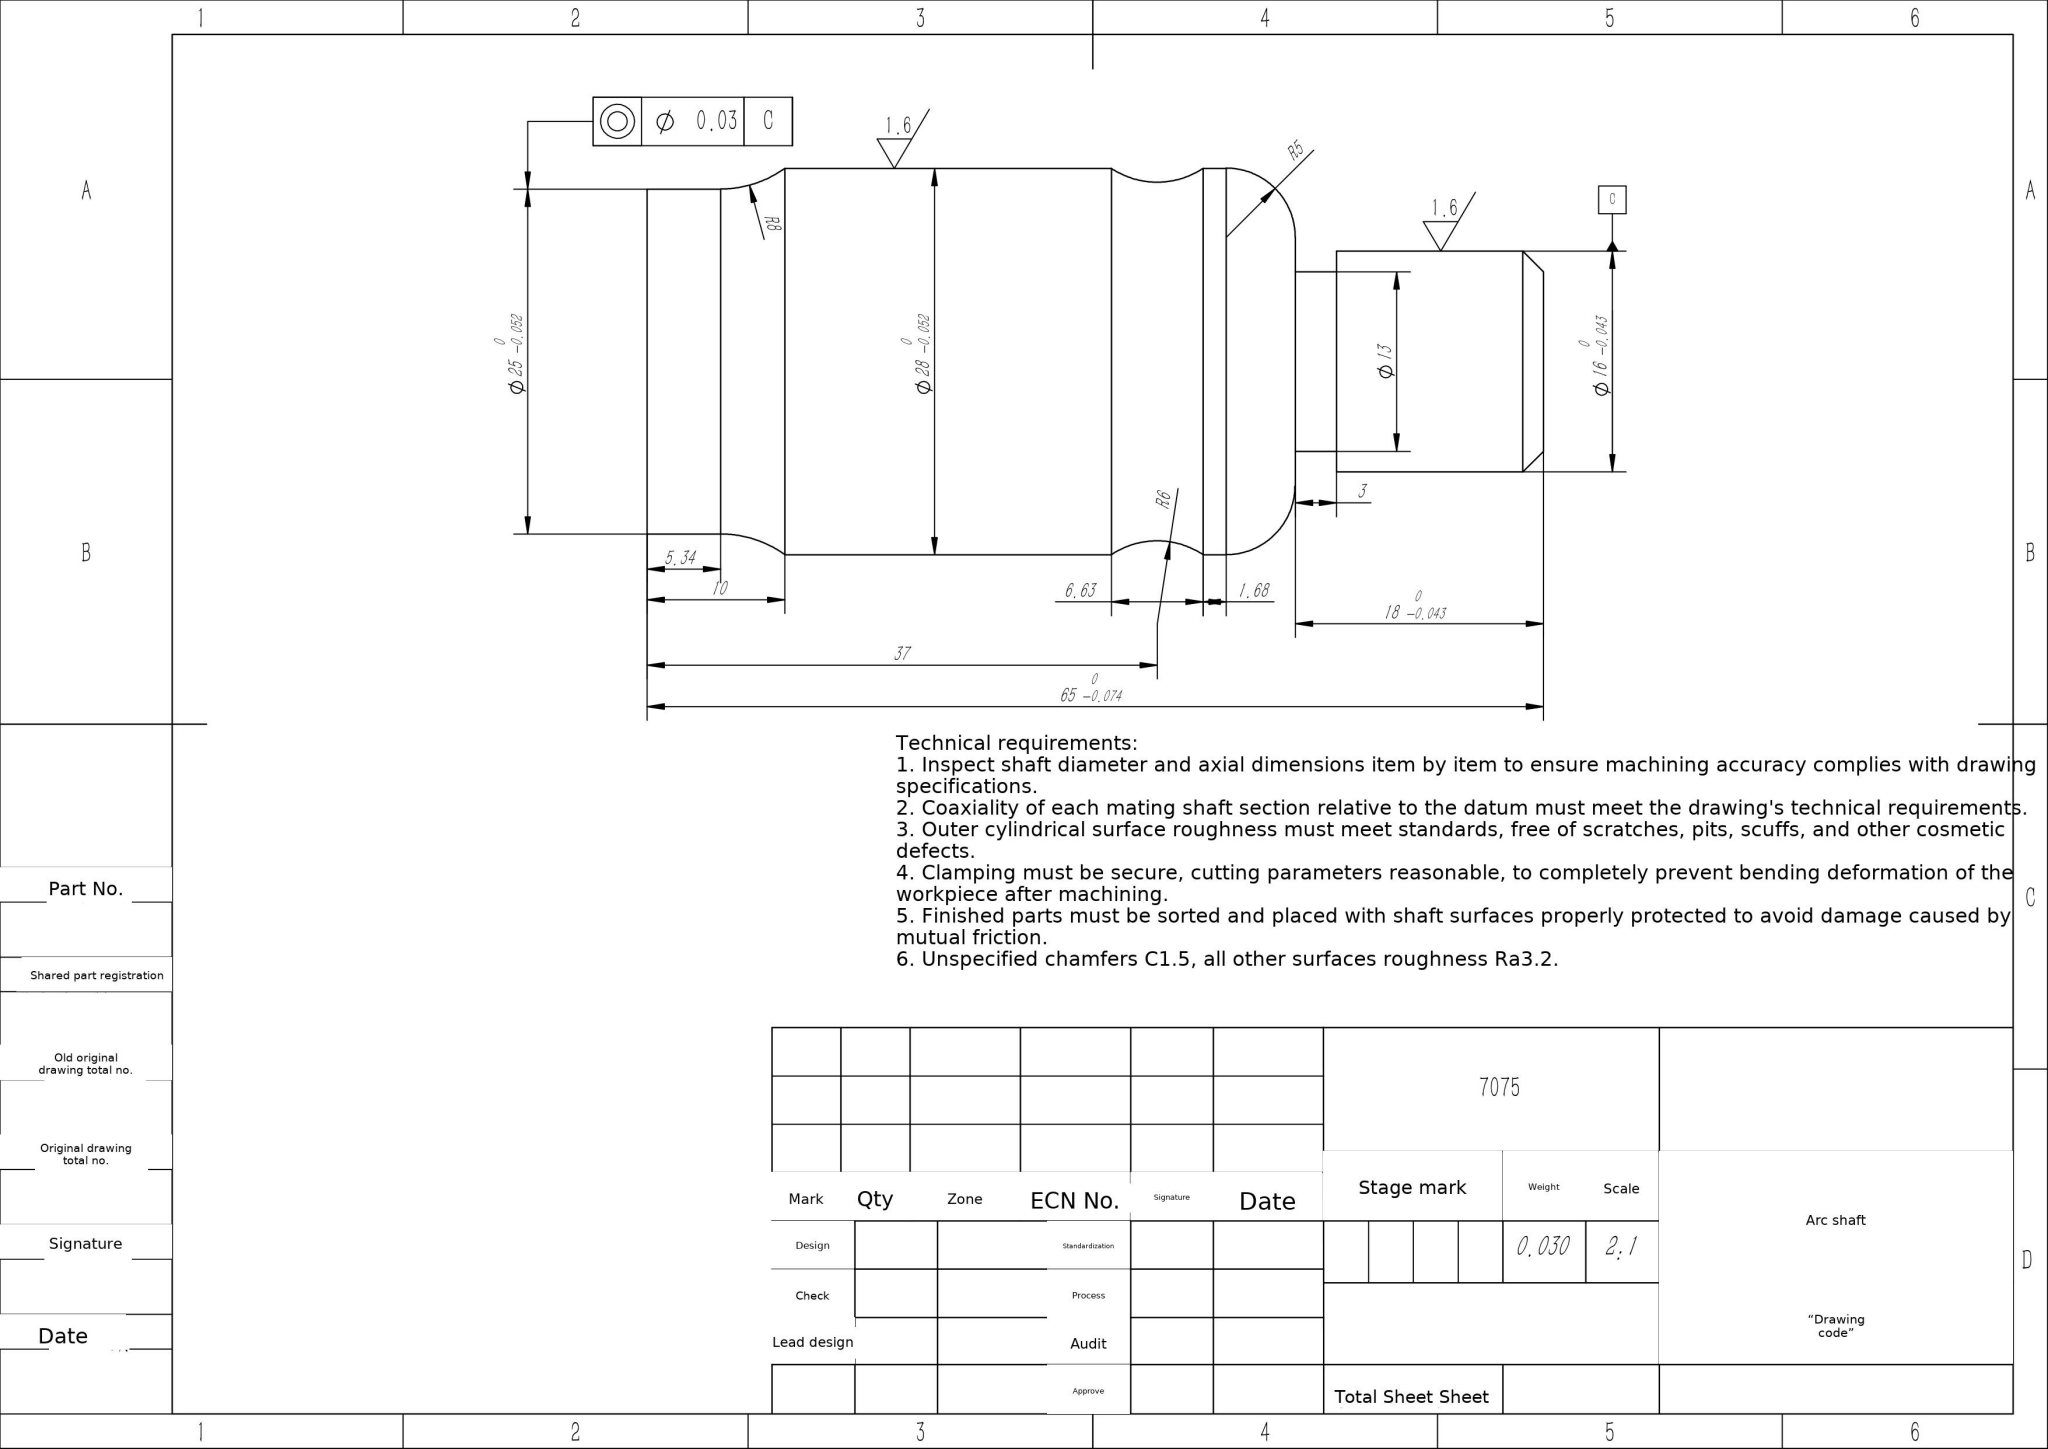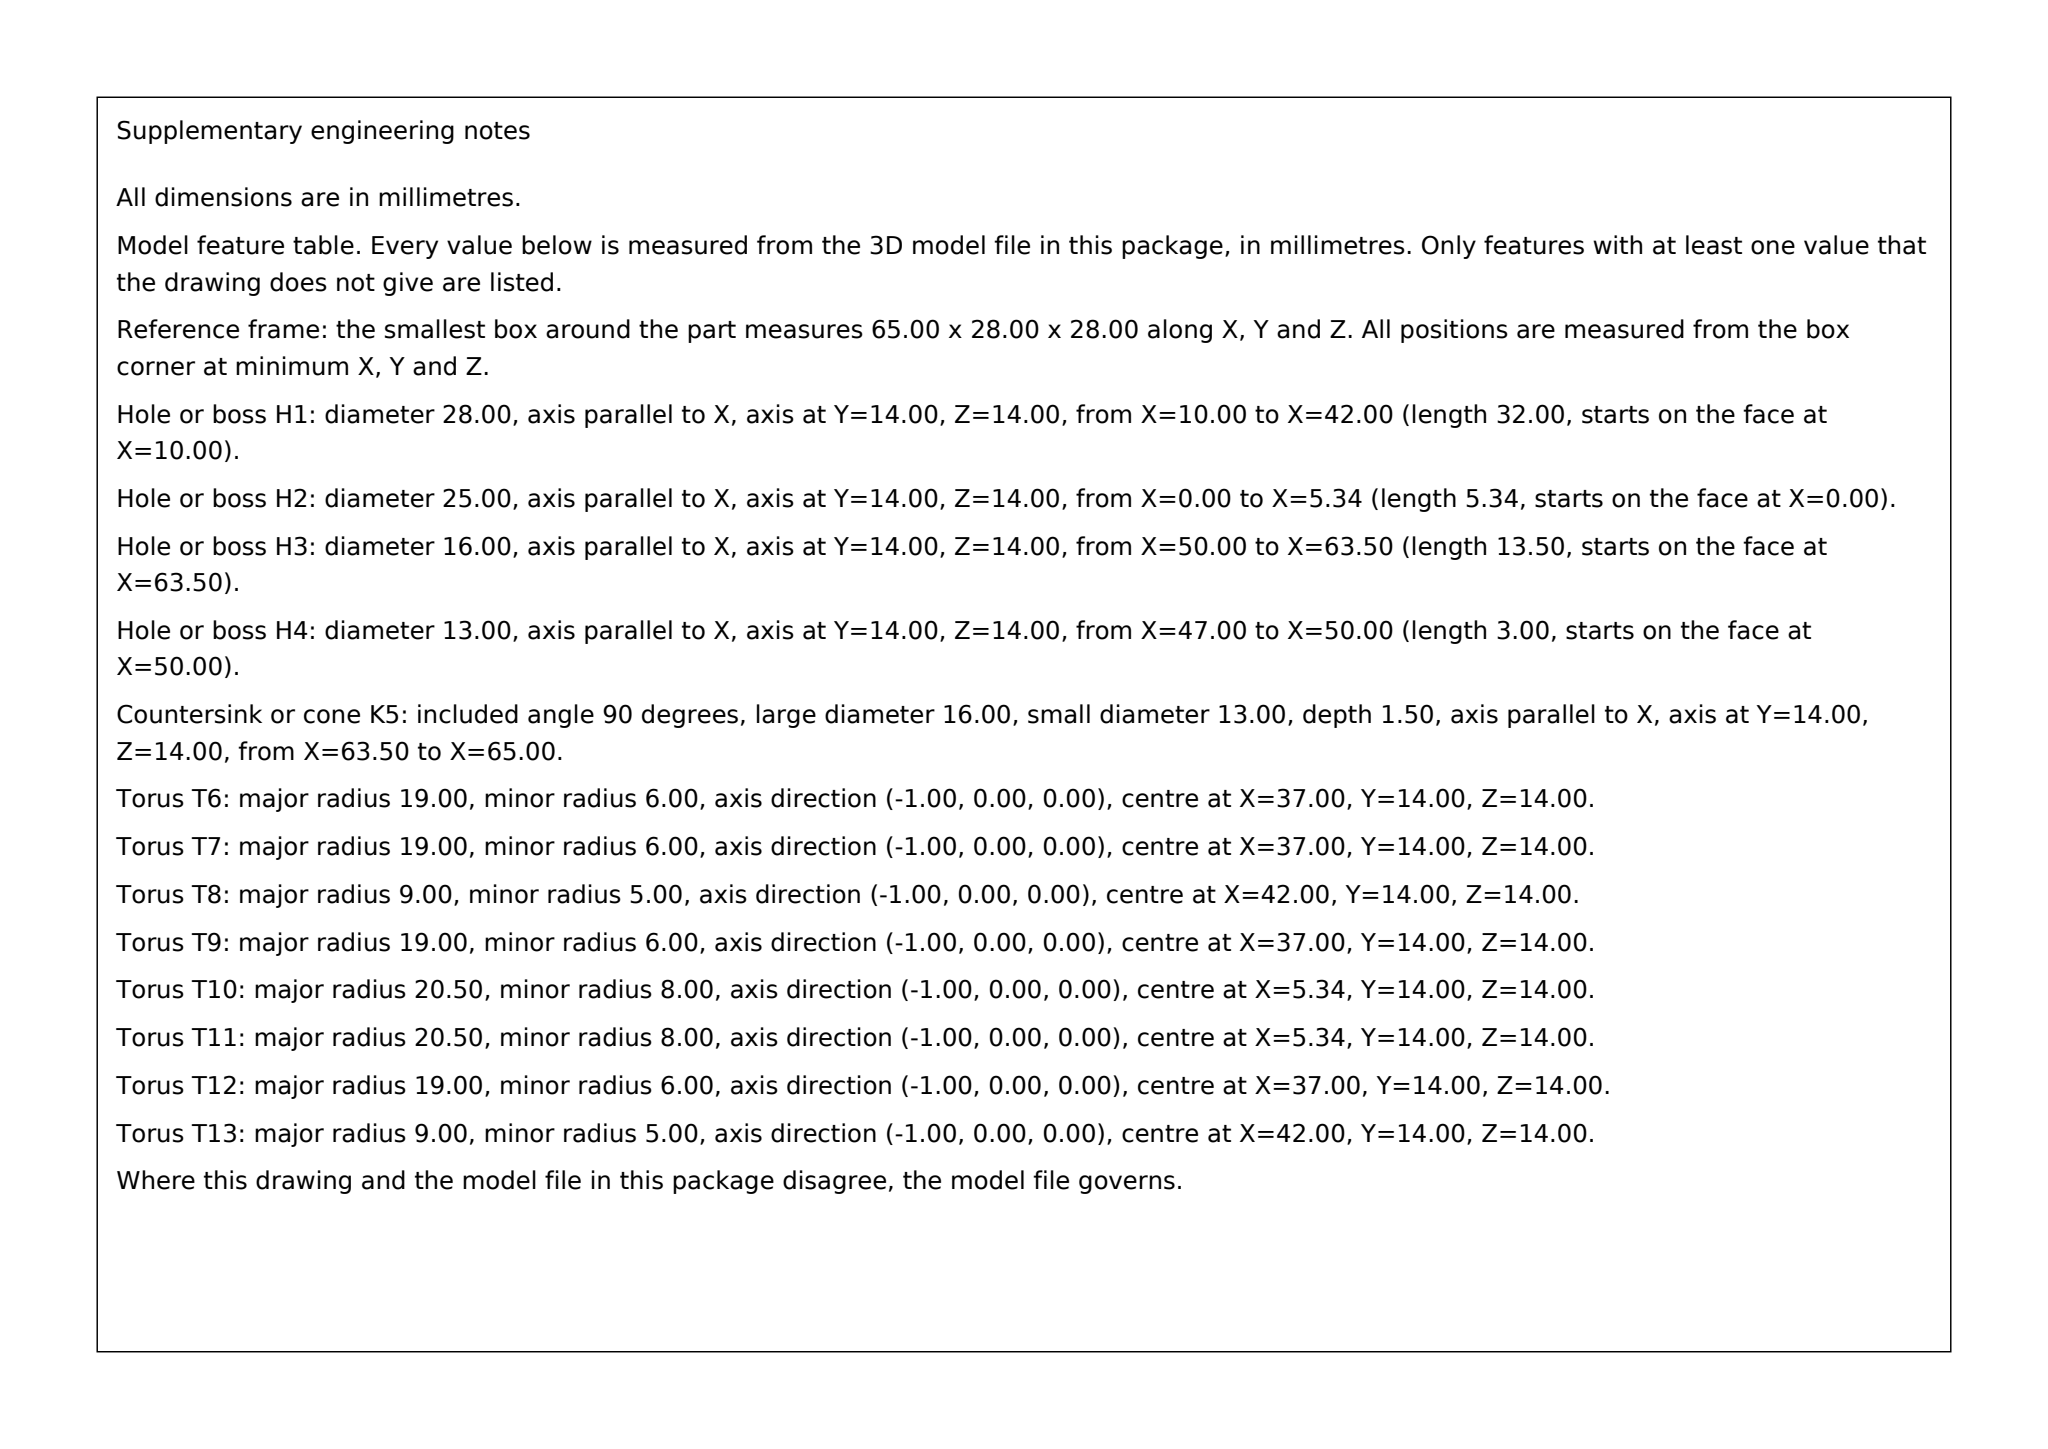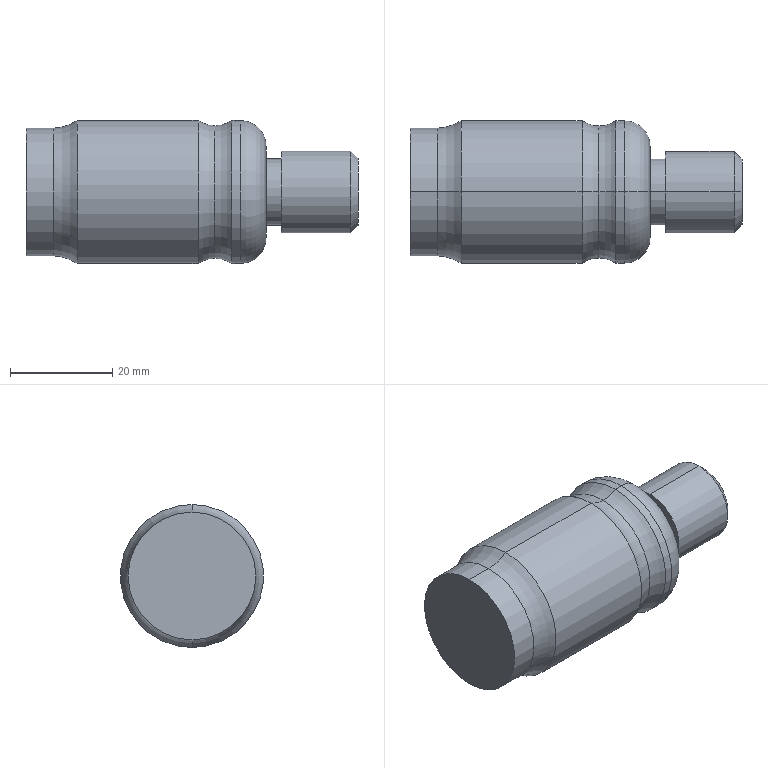Part | SolidWorks | mm | material 7075 | 1 solid | 24 faces | box 65 x 28 x 28 mm | volume 30416 mm3 | cylinder 10 | torus 8 | plane 4 | cone 2 | commonest cylinder face diameters 28 x4 25 x2 16 x2 13 x2
build123d program:
from build123d import *

# Parameters (mm, degrees)
CHAMFER1_SIZE = 1.5


with BuildPart() as part:
    # Model → Revolve1 (revolve)
    with BuildSketch(Plane.XY, mode=Mode.PRIVATE) as revolve1_sk:
        with BuildLine():
            Line((-65.369, 16.383), (-65.369, 3.883))
            Line((-65.369, 3.883), (-0.3693, 3.883))
            Line((-0.3693, 3.883), (-0.3693, 11.883))
            Line((-0.3693, 11.883), (-15.369, 11.883))
            Line((-15.369, 11.883), (-15.369, 10.383))
            Line((-15.369, 10.383), (-18.369, 10.383))
            Line((-18.369, 10.383), (-18.369, 12.883))
            ThreePointArc((-18.369, 12.883), (-19.834, 16.419), (-23.369, 17.883))
            Line((-23.369, 17.883), (-25.053, 17.883))
            ThreePointArc((-25.053, 17.883), (-28.369, 16.883), (-31.686, 17.883))
            Line((-31.686, 17.883), (-55.369, 17.883))
            ThreePointArc((-55.369, 17.883), (-57.584, 16.768), (-60.033, 16.383))
            Line((-60.033, 16.383), (-65.369, 16.383))
        make_face()
    revolve(revolve1_sk.sketch.rotate(Axis((-65.369, 3.883, 0), (1, 0, 0)), 90), axis=Axis((-65.369, 3.883, 0), (1, 0, 0)))

    # Chamfer1
    chamfer1_edges = [part.edges().sort_by_distance(p)[0] for p in [
        (-0.3693, 3.883, -8),
    ]]
    chamfer(chamfer1_edges, length=CHAMFER1_SIZE)


solid = part.part
STEP:
#1=CARTESIAN_POINT('',(-31.686,3.883,14.));
#2=VERTEX_POINT('',#1);
#3=CARTESIAN_POINT('',(-28.369,3.883,13.));
#4=VERTEX_POINT('',#3);
#5=CARTESIAN_POINT('',(-28.369,3.883,19.));
#6=DIRECTION('',(0.,-1.,0.));
#7=DIRECTION('',(0.,0.,-1.));
#8=AXIS2_PLACEMENT_3D('',#5,#6,#7);
#9=CIRCLE('',#8,6.);
#10=EDGE_CURVE('',#2,#4,#9,.T.);
#11=ORIENTED_EDGE('',*,*,#10,.T.);
#12=CARTESIAN_POINT('',(-28.369,3.883,-13.));
#13=VERTEX_POINT('',#12);
#14=CARTESIAN_POINT('',(-28.369,3.883,0.));
#15=DIRECTION('',(-1.,0.,0.));
#16=DIRECTION('',(0.,0.,1.));
#17=AXIS2_PLACEMENT_3D('',#14,#15,#16);
#18=CIRCLE('',#17,13.);
#19=EDGE_CURVE('',#4,#13,#18,.T.);
#20=ORIENTED_EDGE('',*,*,#19,.T.);
#21=CARTESIAN_POINT('',(-31.686,3.883,-14.));
#22=VERTEX_POINT('',#21);
#23=CARTESIAN_POINT('',(-28.369,3.883,-19.));
#24=DIRECTION('',(0.,1.,0.));
#25=DIRECTION('',(0.,-0.,1.));
#26=AXIS2_PLACEMENT_3D('',#23,#24,#25);
#27=CIRCLE('',#26,6.);
#28=EDGE_CURVE('',#22,#13,#27,.T.);
#29=ORIENTED_EDGE('',*,*,#28,.F.);
#30=CARTESIAN_POINT('',(-31.686,3.883,0.));
#31=DIRECTION('',(-1.,0.,0.));
#32=DIRECTION('',(0.,0.,1.));
#33=AXIS2_PLACEMENT_3D('',#30,#31,#32);
#34=CIRCLE('',#33,14.);
#35=EDGE_CURVE('',#2,#22,#34,.T.);
#36=ORIENTED_EDGE('',*,*,#35,.F.);
#37=EDGE_LOOP('',(#11,#20,#29,#36));
#38=FACE_OUTER_BOUND('',#37,.T.);
#39=CARTESIAN_POINT('',(-28.369,3.883,0.));
#40=DIRECTION('',(-1.,0.,0.));
#41=DIRECTION('',(0.,0.,1.));
#42=AXIS2_PLACEMENT_3D('',#39,#40,#41);
#43=TOROIDAL_SURFACE('',#42,19.,6.);
#44=ADVANCED_FACE('',(#38),#43,.F.);
#45=ORIENTED_EDGE('',*,*,#28,.T.);
#46=CARTESIAN_POINT('',(-28.369,3.883,0.));
#47=DIRECTION('',(-1.,0.,0.));
#48=DIRECTION('',(0.,0.,1.));
#49=AXIS2_PLACEMENT_3D('',#46,#47,#48);
#50=CIRCLE('',#49,13.);
#51=EDGE_CURVE('',#13,#4,#50,.T.);
#52=ORIENTED_EDGE('',*,*,#51,.T.);
#53=ORIENTED_EDGE('',*,*,#10,.F.);
#54=CARTESIAN_POINT('',(-31.686,3.883,0.));
#55=DIRECTION('',(-1.,0.,0.));
#56=DIRECTION('',(0.,0.,1.));
#57=AXIS2_PLACEMENT_3D('',#54,#55,#56);
#58=CIRCLE('',#57,14.);
#59=EDGE_CURVE('',#22,#2,#58,.T.);
#60=ORIENTED_EDGE('',*,*,#59,.F.);
#61=EDGE_LOOP('',(#45,#52,#53,#60));
#62=FACE_OUTER_BOUND('',#61,.T.);
#63=CARTESIAN_POINT('',(-28.369,3.883,0.));
#64=DIRECTION('',(-1.,0.,0.));
#65=DIRECTION('',(0.,0.,1.));
#66=AXIS2_PLACEMENT_3D('',#63,#64,#65);
#67=TOROIDAL_SURFACE('',#66,19.,6.);
#68=ADVANCED_FACE('',(#62),#67,.F.);
#69=CARTESIAN_POINT('',(-0.3693,3.883,-6.5));
#70=VERTEX_POINT('',#69);
#71=CARTESIAN_POINT('',(-0.3693,3.883,6.5));
#72=VERTEX_POINT('',#71);
#73=CARTESIAN_POINT('',(-0.3693,3.883,0.));
#74=DIRECTION('',(1.,0.,0.));
#75=DIRECTION('',(0.,0.,1.));
#76=AXIS2_PLACEMENT_3D('',#73,#74,#75);
#77=CIRCLE('',#76,6.5);
#78=EDGE_CURVE('',#70,#72,#77,.T.);
#79=ORIENTED_EDGE('',*,*,#78,.F.);
#80=CARTESIAN_POINT('',(-1.869,3.883,-8.));
#81=VERTEX_POINT('',#80);
#82=CARTESIAN_POINT('',(-1.869,3.883,-8.));
#83=DIRECTION('',(-0.7071,0.,-0.7071));
#84=VECTOR('',#83,1000.);
#85=LINE('',#82,#84);
#86=EDGE_CURVE('',#70,#81,#85,.T.);
#87=ORIENTED_EDGE('',*,*,#86,.T.);
#88=CARTESIAN_POINT('',(-1.869,3.883,8.));
#89=VERTEX_POINT('',#88);
#90=CARTESIAN_POINT('',(-1.869,3.883,0.));
#91=DIRECTION('',(-1.,0.,0.));
#92=DIRECTION('',(0.,0.,1.));
#93=AXIS2_PLACEMENT_3D('',#90,#91,#92);
#94=CIRCLE('',#93,8.);
#95=EDGE_CURVE('',#89,#81,#94,.T.);
#96=ORIENTED_EDGE('',*,*,#95,.F.);
#97=CARTESIAN_POINT('',(-1.869,3.883,8.));
#98=DIRECTION('',(-0.7071,0.,0.7071));
#99=VECTOR('',#98,1000.);
#100=LINE('',#97,#99);
#101=EDGE_CURVE('',#72,#89,#100,.T.);
#102=ORIENTED_EDGE('',*,*,#101,.F.);
#103=EDGE_LOOP('',(#79,#87,#96,#102));
#104=FACE_OUTER_BOUND('',#103,.T.);
#105=CARTESIAN_POINT('',(-1.869,3.883,0.));
#106=DIRECTION('',(-1.,0.,0.));
#107=DIRECTION('',(0.,0.,1.));
#108=AXIS2_PLACEMENT_3D('',#105,#106,#107);
#109=CONICAL_SURFACE('',#108,8.,0.7854);
#110=ADVANCED_FACE('',(#104),#109,.T.);
#111=CARTESIAN_POINT('',(-60.033,3.883,12.5));
#112=VERTEX_POINT('',#111);
#113=CARTESIAN_POINT('',(-60.033,3.883,-12.5));
#114=VERTEX_POINT('',#113);
#115=CARTESIAN_POINT('',(-60.033,3.883,0.));
#116=DIRECTION('',(-1.,0.,0.));
#117=DIRECTION('',(0.,0.,1.));
#118=AXIS2_PLACEMENT_3D('',#115,#116,#117);
#119=CIRCLE('',#118,12.5);
#120=EDGE_CURVE('',#112,#114,#119,.T.);
#121=ORIENTED_EDGE('',*,*,#120,.T.);
#122=CARTESIAN_POINT('',(-65.369,3.883,-12.5));
#123=VERTEX_POINT('',#122);
#124=CARTESIAN_POINT('',(-65.369,3.883,-12.5));
#125=DIRECTION('',(-1.,0.,0.));
#126=VECTOR('',#125,1000.);
#127=LINE('',#124,#126);
#128=EDGE_CURVE('',#114,#123,#127,.T.);
#129=ORIENTED_EDGE('',*,*,#128,.T.);
#130=CARTESIAN_POINT('',(-65.369,3.883,12.5));
#131=VERTEX_POINT('',#130);
#132=CARTESIAN_POINT('',(-65.369,3.883,0.));
#133=DIRECTION('',(-1.,0.,0.));
#134=DIRECTION('',(0.,0.,1.));
#135=AXIS2_PLACEMENT_3D('',#132,#133,#134);
#136=CIRCLE('',#135,12.5);
#137=EDGE_CURVE('',#131,#123,#136,.T.);
#138=ORIENTED_EDGE('',*,*,#137,.F.);
#139=CARTESIAN_POINT('',(-65.369,3.883,12.5));
#140=DIRECTION('',(-1.,0.,0.));
#141=VECTOR('',#140,1000.);
#142=LINE('',#139,#141);
#143=EDGE_CURVE('',#112,#131,#142,.T.);
#144=ORIENTED_EDGE('',*,*,#143,.F.);
#145=EDGE_LOOP('',(#121,#129,#138,#144));
#146=FACE_OUTER_BOUND('',#145,.T.);
#147=CARTESIAN_POINT('',(-65.369,3.883,0.));
#148=DIRECTION('',(-1.,0.,0.));
#149=DIRECTION('',(0.,0.,1.));
#150=AXIS2_PLACEMENT_3D('',#147,#148,#149);
#151=CYLINDRICAL_SURFACE('',#150,12.5);
#152=ADVANCED_FACE('',(#146),#151,.T.);
#153=ORIENTED_EDGE('',*,*,#95,.T.);
#154=CARTESIAN_POINT('',(-15.369,3.883,-8.));
#155=VERTEX_POINT('',#154);
#156=CARTESIAN_POINT('',(-65.369,3.883,-8.));
#157=DIRECTION('',(-1.,0.,0.));
#158=VECTOR('',#157,1000.);
#159=LINE('',#156,#158);
#160=EDGE_CURVE('',#81,#155,#159,.T.);
#161=ORIENTED_EDGE('',*,*,#160,.T.);
#162=CARTESIAN_POINT('',(-15.369,3.883,8.));
#163=VERTEX_POINT('',#162);
#164=CARTESIAN_POINT('',(-15.369,3.883,0.));
#165=DIRECTION('',(-1.,0.,0.));
#166=DIRECTION('',(0.,0.,1.));
#167=AXIS2_PLACEMENT_3D('',#164,#165,#166);
#168=CIRCLE('',#167,8.);
#169=EDGE_CURVE('',#163,#155,#168,.T.);
#170=ORIENTED_EDGE('',*,*,#169,.F.);
#171=CARTESIAN_POINT('',(-65.369,3.883,8.));
#172=DIRECTION('',(-1.,0.,0.));
#173=VECTOR('',#172,1000.);
#174=LINE('',#171,#173);
#175=EDGE_CURVE('',#89,#163,#174,.T.);
#176=ORIENTED_EDGE('',*,*,#175,.F.);
#177=EDGE_LOOP('',(#153,#161,#170,#176));
#178=FACE_OUTER_BOUND('',#177,.T.);
#179=CARTESIAN_POINT('',(-65.369,3.883,0.));
#180=DIRECTION('',(-1.,0.,0.));
#181=DIRECTION('',(0.,0.,1.));
#182=AXIS2_PLACEMENT_3D('',#179,#180,#181);
#183=CYLINDRICAL_SURFACE('',#182,8.);
#184=ADVANCED_FACE('',(#178),#183,.T.);
#185=CARTESIAN_POINT('',(-15.369,3.883,6.5));
#186=VERTEX_POINT('',#185);
#187=CARTESIAN_POINT('',(-15.369,3.883,-6.5));
#188=VERTEX_POINT('',#187);
#189=CARTESIAN_POINT('',(-15.369,3.883,0.));
#190=DIRECTION('',(-1.,0.,0.));
#191=DIRECTION('',(0.,0.,1.));
#192=AXIS2_PLACEMENT_3D('',#189,#190,#191);
#193=CIRCLE('',#192,6.5);
#194=EDGE_CURVE('',#186,#188,#193,.T.);
#195=ORIENTED_EDGE('',*,*,#194,.T.);
#196=CARTESIAN_POINT('',(-18.369,3.883,-6.5));
#197=VERTEX_POINT('',#196);
#198=CARTESIAN_POINT('',(-65.369,3.883,-6.5));
#199=DIRECTION('',(-1.,0.,0.));
#200=VECTOR('',#199,1000.);
#201=LINE('',#198,#200);
#202=EDGE_CURVE('',#188,#197,#201,.T.);
#203=ORIENTED_EDGE('',*,*,#202,.T.);
#204=CARTESIAN_POINT('',(-18.369,3.883,6.5));
#205=VERTEX_POINT('',#204);
#206=CARTESIAN_POINT('',(-18.369,3.883,0.));
#207=DIRECTION('',(-1.,0.,0.));
#208=DIRECTION('',(0.,0.,1.));
#209=AXIS2_PLACEMENT_3D('',#206,#207,#208);
#210=CIRCLE('',#209,6.5);
#211=EDGE_CURVE('',#205,#197,#210,.T.);
#212=ORIENTED_EDGE('',*,*,#211,.F.);
#213=CARTESIAN_POINT('',(-65.369,3.883,6.5));
#214=DIRECTION('',(-1.,0.,0.));
#215=VECTOR('',#214,1000.);
#216=LINE('',#213,#215);
#217=EDGE_CURVE('',#186,#205,#216,.T.);
#218=ORIENTED_EDGE('',*,*,#217,.F.);
#219=EDGE_LOOP('',(#195,#203,#212,#218));
#220=FACE_OUTER_BOUND('',#219,.T.);
#221=CARTESIAN_POINT('',(-65.369,3.883,0.));
#222=DIRECTION('',(-1.,0.,0.));
#223=DIRECTION('',(0.,0.,1.));
#224=AXIS2_PLACEMENT_3D('',#221,#222,#223);
#225=CYLINDRICAL_SURFACE('',#224,6.5);
#226=ADVANCED_FACE('',(#220),#225,.T.);
#227=CARTESIAN_POINT('',(-18.369,3.883,9.));
#228=VERTEX_POINT('',#227);
#229=CARTESIAN_POINT('',(-18.369,3.883,-9.));
#230=VERTEX_POINT('',#229);
#231=CARTESIAN_POINT('',(-18.369,3.883,0.));
#232=DIRECTION('',(-1.,0.,0.));
#233=DIRECTION('',(0.,0.,1.));
#234=AXIS2_PLACEMENT_3D('',#231,#232,#233);
#235=CIRCLE('',#234,9.);
#236=EDGE_CURVE('',#228,#230,#235,.T.);
#237=ORIENTED_EDGE('',*,*,#236,.T.);
#238=CARTESIAN_POINT('',(-23.369,3.883,-14.));
#239=VERTEX_POINT('',#238);
#240=CARTESIAN_POINT('',(-23.369,3.883,-9.));
#241=DIRECTION('',(0.,1.,0.));
#242=DIRECTION('',(0.,-0.,1.));
#243=AXIS2_PLACEMENT_3D('',#240,#241,#242);
#244=CIRCLE('',#243,5.);
#245=EDGE_CURVE('',#230,#239,#244,.T.);
#246=ORIENTED_EDGE('',*,*,#245,.T.);
#247=CARTESIAN_POINT('',(-23.369,3.883,14.));
#248=VERTEX_POINT('',#247);
#249=CARTESIAN_POINT('',(-23.369,3.883,0.));
#250=DIRECTION('',(-1.,0.,0.));
#251=DIRECTION('',(0.,0.,1.));
#252=AXIS2_PLACEMENT_3D('',#249,#250,#251);
#253=CIRCLE('',#252,14.);
#254=EDGE_CURVE('',#248,#239,#253,.T.);
#255=ORIENTED_EDGE('',*,*,#254,.F.);
#256=CARTESIAN_POINT('',(-23.369,3.883,9.));
#257=DIRECTION('',(0.,-1.,0.));
#258=DIRECTION('',(0.,0.,-1.));
#259=AXIS2_PLACEMENT_3D('',#256,#257,#258);
#260=CIRCLE('',#259,5.);
#261=EDGE_CURVE('',#228,#248,#260,.T.);
#262=ORIENTED_EDGE('',*,*,#261,.F.);
#263=EDGE_LOOP('',(#237,#246,#255,#262));
#264=FACE_OUTER_BOUND('',#263,.T.);
#265=CARTESIAN_POINT('',(-23.369,3.883,0.));
#266=DIRECTION('',(-1.,0.,0.));
#267=DIRECTION('',(0.,0.,1.));
#268=AXIS2_PLACEMENT_3D('',#265,#266,#267);
#269=TOROIDAL_SURFACE('',#268,9.,5.);
#270=ADVANCED_FACE('',(#264),#269,.T.);
#271=ORIENTED_EDGE('',*,*,#254,.T.);
#272=CARTESIAN_POINT('',(-25.053,3.883,-14.));
#273=VERTEX_POINT('',#272);
#274=CARTESIAN_POINT('',(-65.369,3.883,-14.));
#275=DIRECTION('',(-1.,0.,0.));
#276=VECTOR('',#275,1000.);
#277=LINE('',#274,#276);
#278=EDGE_CURVE('',#239,#273,#277,.T.);
#279=ORIENTED_EDGE('',*,*,#278,.T.);
#280=CARTESIAN_POINT('',(-25.053,3.883,14.));
#281=VERTEX_POINT('',#280);
#282=CARTESIAN_POINT('',(-25.053,3.883,0.));
#283=DIRECTION('',(-1.,0.,0.));
#284=DIRECTION('',(0.,0.,1.));
#285=AXIS2_PLACEMENT_3D('',#282,#283,#284);
#286=CIRCLE('',#285,14.);
#287=EDGE_CURVE('',#281,#273,#286,.T.);
#288=ORIENTED_EDGE('',*,*,#287,.F.);
#289=CARTESIAN_POINT('',(-65.369,3.883,14.));
#290=DIRECTION('',(-1.,0.,0.));
#291=VECTOR('',#290,1000.);
#292=LINE('',#289,#291);
#293=EDGE_CURVE('',#248,#281,#292,.T.);
#294=ORIENTED_EDGE('',*,*,#293,.F.);
#295=EDGE_LOOP('',(#271,#279,#288,#294));
#296=FACE_OUTER_BOUND('',#295,.T.);
#297=CARTESIAN_POINT('',(-65.369,3.883,0.));
#298=DIRECTION('',(-1.,0.,0.));
#299=DIRECTION('',(0.,0.,1.));
#300=AXIS2_PLACEMENT_3D('',#297,#298,#299);
#301=CYLINDRICAL_SURFACE('',#300,14.);
#302=ADVANCED_FACE('',(#296),#301,.T.);
#303=ORIENTED_EDGE('',*,*,#51,.F.);
#304=CARTESIAN_POINT('',(-28.369,3.883,-19.));
#305=DIRECTION('',(0.,1.,0.));
#306=DIRECTION('',(0.,-0.,1.));
#307=AXIS2_PLACEMENT_3D('',#304,#305,#306);
#308=CIRCLE('',#307,6.);
#309=EDGE_CURVE('',#13,#273,#308,.T.);
#310=ORIENTED_EDGE('',*,*,#309,.T.);
#311=CARTESIAN_POINT('',(-25.053,3.883,0.));
#312=DIRECTION('',(-1.,0.,0.));
#313=DIRECTION('',(0.,0.,1.));
#314=AXIS2_PLACEMENT_3D('',#311,#312,#313);
#315=CIRCLE('',#314,14.);
#316=EDGE_CURVE('',#273,#281,#315,.T.);
#317=ORIENTED_EDGE('',*,*,#316,.T.);
#318=CARTESIAN_POINT('',(-28.369,3.883,19.));
#319=DIRECTION('',(0.,-1.,0.));
#320=DIRECTION('',(0.,0.,-1.));
#321=AXIS2_PLACEMENT_3D('',#318,#319,#320);
#322=CIRCLE('',#321,6.);
#323=EDGE_CURVE('',#4,#281,#322,.T.);
#324=ORIENTED_EDGE('',*,*,#323,.F.);
#325=EDGE_LOOP('',(#303,#310,#317,#324));
#326=FACE_OUTER_BOUND('',#325,.T.);
#327=CARTESIAN_POINT('',(-28.369,3.883,0.));
#328=DIRECTION('',(-1.,0.,0.));
#329=DIRECTION('',(0.,0.,1.));
#330=AXIS2_PLACEMENT_3D('',#327,#328,#329);
#331=TOROIDAL_SURFACE('',#330,19.,6.);
#332=ADVANCED_FACE('',(#326),#331,.F.);
#333=ORIENTED_EDGE('',*,*,#35,.T.);
#334=CARTESIAN_POINT('',(-55.369,3.883,-14.));
#335=VERTEX_POINT('',#334);
#336=CARTESIAN_POINT('',(-65.369,3.883,-14.));
#337=DIRECTION('',(-1.,0.,0.));
#338=VECTOR('',#337,1000.);
#339=LINE('',#336,#338);
#340=EDGE_CURVE('',#22,#335,#339,.T.);
#341=ORIENTED_EDGE('',*,*,#340,.T.);
#342=CARTESIAN_POINT('',(-55.369,3.883,14.));
#343=VERTEX_POINT('',#342);
#344=CARTESIAN_POINT('',(-55.369,3.883,0.));
#345=DIRECTION('',(-1.,0.,0.));
#346=DIRECTION('',(0.,0.,1.));
#347=AXIS2_PLACEMENT_3D('',#344,#345,#346);
#348=CIRCLE('',#347,14.);
#349=EDGE_CURVE('',#343,#335,#348,.T.);
#350=ORIENTED_EDGE('',*,*,#349,.F.);
#351=CARTESIAN_POINT('',(-65.369,3.883,14.));
#352=DIRECTION('',(-1.,0.,0.));
#353=VECTOR('',#352,1000.);
#354=LINE('',#351,#353);
#355=EDGE_CURVE('',#2,#343,#354,.T.);
#356=ORIENTED_EDGE('',*,*,#355,.F.);
#357=EDGE_LOOP('',(#333,#341,#350,#356));
#358=FACE_OUTER_BOUND('',#357,.T.);
#359=CARTESIAN_POINT('',(-65.369,3.883,0.));
#360=DIRECTION('',(-1.,0.,0.));
#361=DIRECTION('',(0.,0.,1.));
#362=AXIS2_PLACEMENT_3D('',#359,#360,#361);
#363=CYLINDRICAL_SURFACE('',#362,14.);
#364=ADVANCED_FACE('',(#358),#363,.T.);
#365=CARTESIAN_POINT('',(-60.033,3.883,0.));
#366=DIRECTION('',(-1.,0.,0.));
#367=DIRECTION('',(0.,0.,1.));
#368=AXIS2_PLACEMENT_3D('',#365,#366,#367);
#369=CIRCLE('',#368,12.5);
#370=EDGE_CURVE('',#114,#112,#369,.T.);
#371=ORIENTED_EDGE('',*,*,#370,.F.);
#372=CARTESIAN_POINT('',(-60.033,3.883,-20.5));
#373=DIRECTION('',(0.,1.,0.));
#374=DIRECTION('',(0.,-0.,1.));
#375=AXIS2_PLACEMENT_3D('',#372,#373,#374);
#376=CIRCLE('',#375,8.);
#377=EDGE_CURVE('',#114,#335,#376,.T.);
#378=ORIENTED_EDGE('',*,*,#377,.T.);
#379=CARTESIAN_POINT('',(-55.369,3.883,0.));
#380=DIRECTION('',(-1.,0.,0.));
#381=DIRECTION('',(0.,0.,1.));
#382=AXIS2_PLACEMENT_3D('',#379,#380,#381);
#383=CIRCLE('',#382,14.);
#384=EDGE_CURVE('',#335,#343,#383,.T.);
#385=ORIENTED_EDGE('',*,*,#384,.T.);
#386=CARTESIAN_POINT('',(-60.033,3.883,20.5));
#387=DIRECTION('',(0.,-1.,0.));
#388=DIRECTION('',(0.,0.,-1.));
#389=AXIS2_PLACEMENT_3D('',#386,#387,#388);
#390=CIRCLE('',#389,8.);
#391=EDGE_CURVE('',#112,#343,#390,.T.);
#392=ORIENTED_EDGE('',*,*,#391,.F.);
#393=EDGE_LOOP('',(#371,#378,#385,#392));
#394=FACE_OUTER_BOUND('',#393,.T.);
#395=CARTESIAN_POINT('',(-60.033,3.883,0.));
#396=DIRECTION('',(-1.,0.,0.));
#397=DIRECTION('',(0.,0.,1.));
#398=AXIS2_PLACEMENT_3D('',#395,#396,#397);
#399=TOROIDAL_SURFACE('',#398,20.5,8.);
#400=ADVANCED_FACE('',(#394),#399,.F.);
#401=ORIENTED_EDGE('',*,*,#377,.F.);
#402=ORIENTED_EDGE('',*,*,#120,.F.);
#403=ORIENTED_EDGE('',*,*,#391,.T.);
#404=ORIENTED_EDGE('',*,*,#349,.T.);
#405=EDGE_LOOP('',(#401,#402,#403,#404));
#406=FACE_OUTER_BOUND('',#405,.T.);
#407=CARTESIAN_POINT('',(-60.033,3.883,0.));
#408=DIRECTION('',(-1.,0.,0.));
#409=DIRECTION('',(0.,0.,1.));
#410=AXIS2_PLACEMENT_3D('',#407,#408,#409);
#411=TOROIDAL_SURFACE('',#410,20.5,8.);
#412=ADVANCED_FACE('',(#406),#411,.F.);
#413=ORIENTED_EDGE('',*,*,#340,.F.);
#414=ORIENTED_EDGE('',*,*,#59,.T.);
#415=ORIENTED_EDGE('',*,*,#355,.T.);
#416=ORIENTED_EDGE('',*,*,#384,.F.);
#417=EDGE_LOOP('',(#413,#414,#415,#416));
#418=FACE_OUTER_BOUND('',#417,.T.);
#419=CARTESIAN_POINT('',(-65.369,3.883,0.));
#420=DIRECTION('',(-1.,0.,0.));
#421=DIRECTION('',(0.,0.,1.));
#422=AXIS2_PLACEMENT_3D('',#419,#420,#421);
#423=CYLINDRICAL_SURFACE('',#422,14.);
#424=ADVANCED_FACE('',(#418),#423,.T.);
#425=ORIENTED_EDGE('',*,*,#19,.F.);
#426=ORIENTED_EDGE('',*,*,#323,.T.);
#427=ORIENTED_EDGE('',*,*,#287,.T.);
#428=ORIENTED_EDGE('',*,*,#309,.F.);
#429=EDGE_LOOP('',(#425,#426,#427,#428));
#430=FACE_OUTER_BOUND('',#429,.T.);
#431=CARTESIAN_POINT('',(-28.369,3.883,0.));
#432=DIRECTION('',(-1.,0.,0.));
#433=DIRECTION('',(0.,0.,1.));
#434=AXIS2_PLACEMENT_3D('',#431,#432,#433);
#435=TOROIDAL_SURFACE('',#434,19.,6.);
#436=ADVANCED_FACE('',(#430),#435,.F.);
#437=ORIENTED_EDGE('',*,*,#278,.F.);
#438=CARTESIAN_POINT('',(-23.369,3.883,0.));
#439=DIRECTION('',(-1.,0.,0.));
#440=DIRECTION('',(0.,0.,1.));
#441=AXIS2_PLACEMENT_3D('',#438,#439,#440);
#442=CIRCLE('',#441,14.);
#443=EDGE_CURVE('',#239,#248,#442,.T.);
#444=ORIENTED_EDGE('',*,*,#443,.T.);
#445=ORIENTED_EDGE('',*,*,#293,.T.);
#446=ORIENTED_EDGE('',*,*,#316,.F.);
#447=EDGE_LOOP('',(#437,#444,#445,#446));
#448=FACE_OUTER_BOUND('',#447,.T.);
#449=CARTESIAN_POINT('',(-65.369,3.883,0.));
#450=DIRECTION('',(-1.,0.,0.));
#451=DIRECTION('',(0.,0.,1.));
#452=AXIS2_PLACEMENT_3D('',#449,#450,#451);
#453=CYLINDRICAL_SURFACE('',#452,14.);
#454=ADVANCED_FACE('',(#448),#453,.T.);
#455=ORIENTED_EDGE('',*,*,#245,.F.);
#456=CARTESIAN_POINT('',(-18.369,3.883,0.));
#457=DIRECTION('',(-1.,0.,0.));
#458=DIRECTION('',(0.,0.,1.));
#459=AXIS2_PLACEMENT_3D('',#456,#457,#458);
#460=CIRCLE('',#459,9.);
#461=EDGE_CURVE('',#230,#228,#460,.T.);
#462=ORIENTED_EDGE('',*,*,#461,.T.);
#463=ORIENTED_EDGE('',*,*,#261,.T.);
#464=ORIENTED_EDGE('',*,*,#443,.F.);
#465=EDGE_LOOP('',(#455,#462,#463,#464));
#466=FACE_OUTER_BOUND('',#465,.T.);
#467=CARTESIAN_POINT('',(-23.369,3.883,0.));
#468=DIRECTION('',(-1.,0.,0.));
#469=DIRECTION('',(0.,0.,1.));
#470=AXIS2_PLACEMENT_3D('',#467,#468,#469);
#471=TOROIDAL_SURFACE('',#470,9.,5.);
#472=ADVANCED_FACE('',(#466),#471,.T.);
#473=ORIENTED_EDGE('',*,*,#236,.F.);
#474=ORIENTED_EDGE('',*,*,#461,.F.);
#475=EDGE_LOOP('',(#473,#474));
#476=FACE_OUTER_BOUND('',#475,.T.);
#477=ORIENTED_EDGE('',*,*,#211,.T.);
#478=CARTESIAN_POINT('',(-18.369,3.883,0.));
#479=DIRECTION('',(-1.,0.,0.));
#480=DIRECTION('',(0.,0.,1.));
#481=AXIS2_PLACEMENT_3D('',#478,#479,#480);
#482=CIRCLE('',#481,6.5);
#483=EDGE_CURVE('',#197,#205,#482,.T.);
#484=ORIENTED_EDGE('',*,*,#483,.T.);
#485=EDGE_LOOP('',(#477,#484));
#486=FACE_BOUND('',#485,.T.);
#487=CARTESIAN_POINT('',(-18.369,12.883,0.));
#488=DIRECTION('',(-1.,0.,0.));
#489=DIRECTION('',(0.,0.,1.));
#490=AXIS2_PLACEMENT_3D('',#487,#488,#489);
#491=PLANE('',#490);
#492=ADVANCED_FACE('',(#476,#486),#491,.F.);
#493=ORIENTED_EDGE('',*,*,#202,.F.);
#494=CARTESIAN_POINT('',(-15.369,3.883,0.));
#495=DIRECTION('',(-1.,0.,0.));
#496=DIRECTION('',(0.,0.,1.));
#497=AXIS2_PLACEMENT_3D('',#494,#495,#496);
#498=CIRCLE('',#497,6.5);
#499=EDGE_CURVE('',#188,#186,#498,.T.);
#500=ORIENTED_EDGE('',*,*,#499,.T.);
#501=ORIENTED_EDGE('',*,*,#217,.T.);
#502=ORIENTED_EDGE('',*,*,#483,.F.);
#503=EDGE_LOOP('',(#493,#500,#501,#502));
#504=FACE_OUTER_BOUND('',#503,.T.);
#505=CARTESIAN_POINT('',(-65.369,3.883,0.));
#506=DIRECTION('',(-1.,0.,0.));
#507=DIRECTION('',(0.,0.,1.));
#508=AXIS2_PLACEMENT_3D('',#505,#506,#507);
#509=CYLINDRICAL_SURFACE('',#508,6.5);
#510=ADVANCED_FACE('',(#504),#509,.T.);
#511=ORIENTED_EDGE('',*,*,#194,.F.);
#512=ORIENTED_EDGE('',*,*,#499,.F.);
#513=EDGE_LOOP('',(#511,#512));
#514=FACE_BOUND('',#513,.T.);
#515=ORIENTED_EDGE('',*,*,#169,.T.);
#516=CARTESIAN_POINT('',(-15.369,3.883,0.));
#517=DIRECTION('',(-1.,0.,0.));
#518=DIRECTION('',(0.,0.,1.));
#519=AXIS2_PLACEMENT_3D('',#516,#517,#518);
#520=CIRCLE('',#519,8.);
#521=EDGE_CURVE('',#155,#163,#520,.T.);
#522=ORIENTED_EDGE('',*,*,#521,.T.);
#523=EDGE_LOOP('',(#515,#522));
#524=FACE_OUTER_BOUND('',#523,.T.);
#525=CARTESIAN_POINT('',(-15.369,10.383,0.));
#526=DIRECTION('',(1.,0.,0.));
#527=DIRECTION('',(0.,0.,-1.));
#528=AXIS2_PLACEMENT_3D('',#525,#526,#527);
#529=PLANE('',#528);
#530=ADVANCED_FACE('',(#514,#524),#529,.F.);
#531=ORIENTED_EDGE('',*,*,#160,.F.);
#532=CARTESIAN_POINT('',(-1.869,3.883,0.));
#533=DIRECTION('',(-1.,0.,0.));
#534=DIRECTION('',(0.,0.,1.));
#535=AXIS2_PLACEMENT_3D('',#532,#533,#534);
#536=CIRCLE('',#535,8.);
#537=EDGE_CURVE('',#81,#89,#536,.T.);
#538=ORIENTED_EDGE('',*,*,#537,.T.);
#539=ORIENTED_EDGE('',*,*,#175,.T.);
#540=ORIENTED_EDGE('',*,*,#521,.F.);
#541=EDGE_LOOP('',(#531,#538,#539,#540));
#542=FACE_OUTER_BOUND('',#541,.T.);
#543=CARTESIAN_POINT('',(-65.369,3.883,0.));
#544=DIRECTION('',(-1.,0.,0.));
#545=DIRECTION('',(0.,0.,1.));
#546=AXIS2_PLACEMENT_3D('',#543,#544,#545);
#547=CYLINDRICAL_SURFACE('',#546,8.);
#548=ADVANCED_FACE('',(#542),#547,.T.);
#549=CARTESIAN_POINT('',(-0.3693,3.883,0.));
#550=DIRECTION('',(1.,0.,0.));
#551=DIRECTION('',(0.,0.,1.));
#552=AXIS2_PLACEMENT_3D('',#549,#550,#551);
#553=CIRCLE('',#552,6.5);
#554=EDGE_CURVE('',#72,#70,#553,.T.);
#555=ORIENTED_EDGE('',*,*,#554,.T.);
#556=ORIENTED_EDGE('',*,*,#78,.T.);
#557=EDGE_LOOP('',(#555,#556));
#558=FACE_OUTER_BOUND('',#557,.T.);
#559=CARTESIAN_POINT('',(-0.3693,11.883,0.));
#560=DIRECTION('',(-1.,0.,0.));
#561=DIRECTION('',(0.,0.,1.));
#562=AXIS2_PLACEMENT_3D('',#559,#560,#561);
#563=PLANE('',#562);
#564=ADVANCED_FACE('',(#558),#563,.F.);
#565=ORIENTED_EDGE('',*,*,#137,.T.);
#566=CARTESIAN_POINT('',(-65.369,3.883,0.));
#567=DIRECTION('',(-1.,0.,0.));
#568=DIRECTION('',(0.,0.,1.));
#569=AXIS2_PLACEMENT_3D('',#566,#567,#568);
#570=CIRCLE('',#569,12.5);
#571=EDGE_CURVE('',#123,#131,#570,.T.);
#572=ORIENTED_EDGE('',*,*,#571,.T.);
#573=EDGE_LOOP('',(#565,#572));
#574=FACE_OUTER_BOUND('',#573,.T.);
#575=CARTESIAN_POINT('',(-65.369,16.383,0.));
#576=DIRECTION('',(1.,0.,0.));
#577=DIRECTION('',(0.,0.,-1.));
#578=AXIS2_PLACEMENT_3D('',#575,#576,#577);
#579=PLANE('',#578);
#580=ADVANCED_FACE('',(#574),#579,.F.);
#581=ORIENTED_EDGE('',*,*,#128,.F.);
#582=ORIENTED_EDGE('',*,*,#370,.T.);
#583=ORIENTED_EDGE('',*,*,#143,.T.);
#584=ORIENTED_EDGE('',*,*,#571,.F.);
#585=EDGE_LOOP('',(#581,#582,#583,#584));
#586=FACE_OUTER_BOUND('',#585,.T.);
#587=CARTESIAN_POINT('',(-65.369,3.883,0.));
#588=DIRECTION('',(-1.,0.,0.));
#589=DIRECTION('',(0.,0.,1.));
#590=AXIS2_PLACEMENT_3D('',#587,#588,#589);
#591=CYLINDRICAL_SURFACE('',#590,12.5);
#592=ADVANCED_FACE('',(#586),#591,.T.);
#593=ORIENTED_EDGE('',*,*,#86,.F.);
#594=ORIENTED_EDGE('',*,*,#554,.F.);
#595=ORIENTED_EDGE('',*,*,#101,.T.);
#596=ORIENTED_EDGE('',*,*,#537,.F.);
#597=EDGE_LOOP('',(#593,#594,#595,#596));
#598=FACE_OUTER_BOUND('',#597,.T.);
#599=CARTESIAN_POINT('',(-1.869,3.883,0.));
#600=DIRECTION('',(-1.,0.,0.));
#601=DIRECTION('',(0.,0.,1.));
#602=AXIS2_PLACEMENT_3D('',#599,#600,#601);
#603=CONICAL_SURFACE('',#602,8.,0.7854);
#604=ADVANCED_FACE('',(#598),#603,.T.);
#605=CLOSED_SHELL('',(#44,#68,#110,#152,#184,#226,#270,#302,#332,#364,#400,#412,#424,#436,#454,#472,#492,#510,#530,#548,#564,#580,#592,#604));
#606=MANIFOLD_SOLID_BREP('',#605);
#607=CARTESIAN_POINT('',(0.,0.,0.));
#608=DIRECTION('',(0.,0.,1.));
#609=DIRECTION('',(1.,0.,0.));
#610=AXIS2_PLACEMENT_3D('',#607,#608,#609);
#611=(LENGTH_UNIT()NAMED_UNIT(*)SI_UNIT(.MILLI.,.METRE.));
#612=UNCERTAINTY_MEASURE_WITH_UNIT(LENGTH_MEASURE(0.00001),#611,'','');
#613=(NAMED_UNIT(*)PLANE_ANGLE_UNIT()SI_UNIT($,.RADIAN.));
#614=(NAMED_UNIT(*)SI_UNIT($,.STERADIAN.)SOLID_ANGLE_UNIT());
#615=(GEOMETRIC_REPRESENTATION_CONTEXT(3)GLOBAL_UNCERTAINTY_ASSIGNED_CONTEXT((#612))GLOBAL_UNIT_ASSIGNED_CONTEXT((#611,#613,#614))REPRESENTATION_CONTEXT('',''));
#616=ADVANCED_BREP_SHAPE_REPRESENTATION('',(#606,#610),#615);